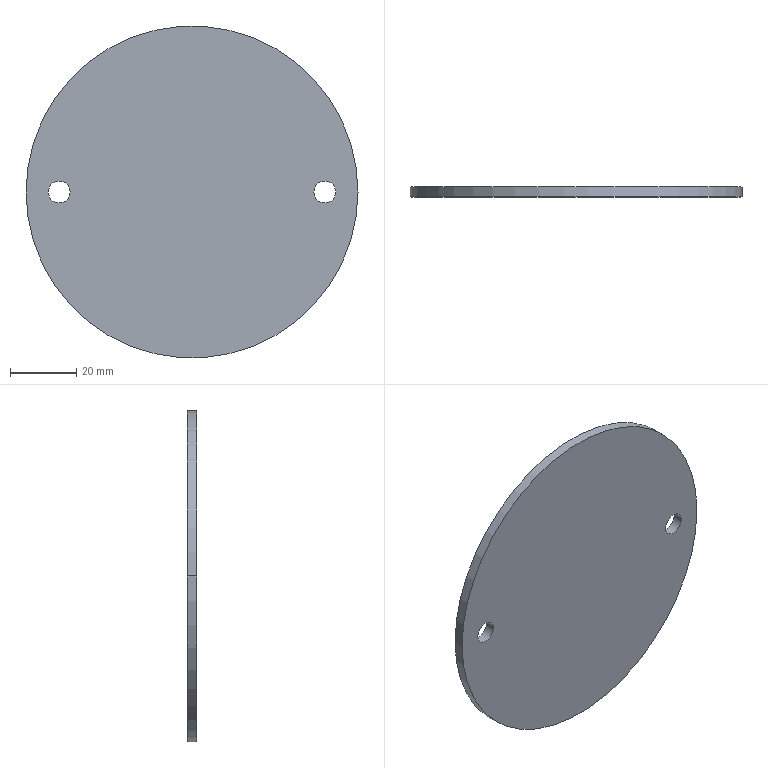Component | SolidWorks | YC1-250-04BalancerAssembly#16673-1_YC1-250-04-09Cover-1 | 1 solid | 8 faces | box 100 x 3 x 100 mm | volume 23357 mm3 | cylinder 6 | plane 2 | commonest cylinder face diameters 6.6 x4 100 x2 | material Plain Carbon Steel
STEP:
#1=COLOUR_RGB('',0.7922,0.8196,0.9333);
#2=FILL_AREA_STYLE_COLOUR('',#1);
#3=FILL_AREA_STYLE('',(#2));
#4=SURFACE_STYLE_FILL_AREA(#3);
#5=SURFACE_SIDE_STYLE('',(#4));
#6=SURFACE_STYLE_USAGE(.BOTH.,#5);
#7=PRESENTATION_STYLE_ASSIGNMENT((#6));
#8=CARTESIAN_POINT('',(-16.142,180.157,-0.));
#9=VERTEX_POINT('',#8);
#10=CARTESIAN_POINT('',(-20.079,180.157,-0.));
#11=VERTEX_POINT('',#10);
#12=CARTESIAN_POINT('',(-18.11,180.157,-0.));
#13=DIRECTION('',(-0.,1.,-0.));
#14=DIRECTION('',(-1.,0.,0.));
#15=AXIS2_PLACEMENT_3D('',#12,#13,#14);
#16=CIRCLE('',#15,1.969);
#17=EDGE_CURVE('',#9,#11,#16,.T.);
#18=ORIENTED_EDGE('',*,*,#17,.F.);
#19=CARTESIAN_POINT('',(-16.142,180.039,-0.));
#20=VERTEX_POINT('',#19);
#21=CARTESIAN_POINT('',(-16.142,180.157,-0.));
#22=DIRECTION('',(0.,-1.,0.));
#23=VECTOR('',#22,39.37);
#24=LINE('',#21,#23);
#25=EDGE_CURVE('',#9,#20,#24,.T.);
#26=ORIENTED_EDGE('',*,*,#25,.T.);
#27=CARTESIAN_POINT('',(-20.079,180.039,-0.));
#28=VERTEX_POINT('',#27);
#29=CARTESIAN_POINT('',(-18.11,180.039,-0.));
#30=DIRECTION('',(-0.,1.,-0.));
#31=DIRECTION('',(-1.,0.,0.));
#32=AXIS2_PLACEMENT_3D('',#29,#30,#31);
#33=CIRCLE('',#32,1.969);
#34=EDGE_CURVE('',#20,#28,#33,.T.);
#35=ORIENTED_EDGE('',*,*,#34,.T.);
#36=CARTESIAN_POINT('',(-20.079,180.157,-0.));
#37=DIRECTION('',(0.,-1.,0.));
#38=VECTOR('',#37,39.37);
#39=LINE('',#36,#38);
#40=EDGE_CURVE('',#11,#28,#39,.T.);
#41=ORIENTED_EDGE('',*,*,#40,.F.);
#42=EDGE_LOOP('',(#18,#26,#35,#41));
#43=FACE_OUTER_BOUND('',#42,.T.);
#44=CARTESIAN_POINT('',(-18.11,180.157,-0.));
#45=DIRECTION('',(0.,-1.,0.));
#46=DIRECTION('',(-1.,0.,0.));
#47=AXIS2_PLACEMENT_3D('',#44,#45,#46);
#48=CYLINDRICAL_SURFACE('',#47,1.969);
#49=ADVANCED_FACE('',(#43),#48,.T.);
#50=CARTESIAN_POINT('',(-16.665,180.039,-0.));
#51=VERTEX_POINT('',#50);
#52=CARTESIAN_POINT('',(-16.406,180.039,-0.));
#53=VERTEX_POINT('',#52);
#54=CARTESIAN_POINT('',(-16.535,180.039,-0.));
#55=DIRECTION('',(-0.,1.,-0.));
#56=DIRECTION('',(1.,0.,-0.));
#57=AXIS2_PLACEMENT_3D('',#54,#55,#56);
#58=CIRCLE('',#57,0.1299);
#59=EDGE_CURVE('',#51,#53,#58,.T.);
#60=ORIENTED_EDGE('',*,*,#59,.F.);
#61=CARTESIAN_POINT('',(-16.665,180.157,-0.));
#62=VERTEX_POINT('',#61);
#63=CARTESIAN_POINT('',(-16.665,180.157,-0.));
#64=DIRECTION('',(-0.,1.,-0.));
#65=VECTOR('',#64,39.37);
#66=LINE('',#63,#65);
#67=EDGE_CURVE('',#51,#62,#66,.T.);
#68=ORIENTED_EDGE('',*,*,#67,.T.);
#69=CARTESIAN_POINT('',(-16.406,180.157,-0.));
#70=VERTEX_POINT('',#69);
#71=CARTESIAN_POINT('',(-16.535,180.157,-0.));
#72=DIRECTION('',(0.,-1.,0.));
#73=DIRECTION('',(1.,0.,-0.));
#74=AXIS2_PLACEMENT_3D('',#71,#72,#73);
#75=CIRCLE('',#74,0.1299);
#76=EDGE_CURVE('',#70,#62,#75,.T.);
#77=ORIENTED_EDGE('',*,*,#76,.F.);
#78=CARTESIAN_POINT('',(-16.406,180.157,-0.));
#79=DIRECTION('',(-0.,1.,-0.));
#80=VECTOR('',#79,39.37);
#81=LINE('',#78,#80);
#82=EDGE_CURVE('',#53,#70,#81,.T.);
#83=ORIENTED_EDGE('',*,*,#82,.F.);
#84=EDGE_LOOP('',(#60,#68,#77,#83));
#85=FACE_OUTER_BOUND('',#84,.T.);
#86=CARTESIAN_POINT('',(-16.535,180.157,-0.));
#87=DIRECTION('',(-0.,1.,-0.));
#88=DIRECTION('',(1.,0.,-0.));
#89=AXIS2_PLACEMENT_3D('',#86,#87,#88);
#90=CYLINDRICAL_SURFACE('',#89,0.1299);
#91=ADVANCED_FACE('',(#85),#90,.F.);
#92=CARTESIAN_POINT('',(-19.815,180.039,-0.));
#93=VERTEX_POINT('',#92);
#94=CARTESIAN_POINT('',(-19.555,180.039,-0.));
#95=VERTEX_POINT('',#94);
#96=CARTESIAN_POINT('',(-19.685,180.039,-0.));
#97=DIRECTION('',(-0.,1.,-0.));
#98=DIRECTION('',(1.,0.,-0.));
#99=AXIS2_PLACEMENT_3D('',#96,#97,#98);
#100=CIRCLE('',#99,0.1299);
#101=EDGE_CURVE('',#93,#95,#100,.T.);
#102=ORIENTED_EDGE('',*,*,#101,.F.);
#103=CARTESIAN_POINT('',(-19.815,180.157,-0.));
#104=VERTEX_POINT('',#103);
#105=CARTESIAN_POINT('',(-19.815,180.157,-0.));
#106=DIRECTION('',(-0.,1.,-0.));
#107=VECTOR('',#106,39.37);
#108=LINE('',#105,#107);
#109=EDGE_CURVE('',#93,#104,#108,.T.);
#110=ORIENTED_EDGE('',*,*,#109,.T.);
#111=CARTESIAN_POINT('',(-19.555,180.157,-0.));
#112=VERTEX_POINT('',#111);
#113=CARTESIAN_POINT('',(-19.685,180.157,-0.));
#114=DIRECTION('',(0.,-1.,0.));
#115=DIRECTION('',(1.,0.,-0.));
#116=AXIS2_PLACEMENT_3D('',#113,#114,#115);
#117=CIRCLE('',#116,0.1299);
#118=EDGE_CURVE('',#112,#104,#117,.T.);
#119=ORIENTED_EDGE('',*,*,#118,.F.);
#120=CARTESIAN_POINT('',(-19.555,180.157,-0.));
#121=DIRECTION('',(-0.,1.,-0.));
#122=VECTOR('',#121,39.37);
#123=LINE('',#120,#122);
#124=EDGE_CURVE('',#95,#112,#123,.T.);
#125=ORIENTED_EDGE('',*,*,#124,.F.);
#126=EDGE_LOOP('',(#102,#110,#119,#125));
#127=FACE_OUTER_BOUND('',#126,.T.);
#128=CARTESIAN_POINT('',(-19.685,180.157,-0.));
#129=DIRECTION('',(-0.,1.,-0.));
#130=DIRECTION('',(1.,0.,-0.));
#131=AXIS2_PLACEMENT_3D('',#128,#129,#130);
#132=CYLINDRICAL_SURFACE('',#131,0.1299);
#133=ADVANCED_FACE('',(#127),#132,.F.);
#134=CARTESIAN_POINT('',(-18.11,180.157,-0.));
#135=DIRECTION('',(-0.,1.,-0.));
#136=DIRECTION('',(-1.,0.,0.));
#137=AXIS2_PLACEMENT_3D('',#134,#135,#136);
#138=CIRCLE('',#137,1.969);
#139=EDGE_CURVE('',#11,#9,#138,.T.);
#140=ORIENTED_EDGE('',*,*,#139,.T.);
#141=ORIENTED_EDGE('',*,*,#17,.T.);
#142=EDGE_LOOP('',(#140,#141));
#143=FACE_OUTER_BOUND('',#142,.T.);
#144=ORIENTED_EDGE('',*,*,#76,.T.);
#145=CARTESIAN_POINT('',(-16.535,180.157,-0.));
#146=DIRECTION('',(0.,-1.,0.));
#147=DIRECTION('',(1.,0.,-0.));
#148=AXIS2_PLACEMENT_3D('',#145,#146,#147);
#149=CIRCLE('',#148,0.1299);
#150=EDGE_CURVE('',#62,#70,#149,.T.);
#151=ORIENTED_EDGE('',*,*,#150,.T.);
#152=EDGE_LOOP('',(#144,#151));
#153=FACE_BOUND('',#152,.T.);
#154=ORIENTED_EDGE('',*,*,#118,.T.);
#155=CARTESIAN_POINT('',(-19.685,180.157,-0.));
#156=DIRECTION('',(0.,-1.,0.));
#157=DIRECTION('',(1.,0.,-0.));
#158=AXIS2_PLACEMENT_3D('',#155,#156,#157);
#159=CIRCLE('',#158,0.1299);
#160=EDGE_CURVE('',#104,#112,#159,.T.);
#161=ORIENTED_EDGE('',*,*,#160,.T.);
#162=EDGE_LOOP('',(#154,#161));
#163=FACE_BOUND('',#162,.T.);
#164=CARTESIAN_POINT('',(-18.11,180.157,-0.));
#165=DIRECTION('',(-0.,1.,-0.));
#166=DIRECTION('',(1.,0.,-0.));
#167=AXIS2_PLACEMENT_3D('',#164,#165,#166);
#168=PLANE('',#167);
#169=ADVANCED_FACE('',(#143,#153,#163),#168,.T.);
#170=ORIENTED_EDGE('',*,*,#25,.F.);
#171=ORIENTED_EDGE('',*,*,#139,.F.);
#172=ORIENTED_EDGE('',*,*,#40,.T.);
#173=CARTESIAN_POINT('',(-18.11,180.039,-0.));
#174=DIRECTION('',(-0.,1.,-0.));
#175=DIRECTION('',(-1.,0.,0.));
#176=AXIS2_PLACEMENT_3D('',#173,#174,#175);
#177=CIRCLE('',#176,1.969);
#178=EDGE_CURVE('',#28,#20,#177,.T.);
#179=ORIENTED_EDGE('',*,*,#178,.T.);
#180=EDGE_LOOP('',(#170,#171,#172,#179));
#181=FACE_OUTER_BOUND('',#180,.T.);
#182=CARTESIAN_POINT('',(-18.11,180.157,-0.));
#183=DIRECTION('',(0.,-1.,0.));
#184=DIRECTION('',(-1.,0.,0.));
#185=AXIS2_PLACEMENT_3D('',#182,#183,#184);
#186=CYLINDRICAL_SURFACE('',#185,1.969);
#187=ADVANCED_FACE('',(#181),#186,.T.);
#188=ORIENTED_EDGE('',*,*,#67,.F.);
#189=CARTESIAN_POINT('',(-16.535,180.039,-0.));
#190=DIRECTION('',(-0.,1.,-0.));
#191=DIRECTION('',(1.,0.,-0.));
#192=AXIS2_PLACEMENT_3D('',#189,#190,#191);
#193=CIRCLE('',#192,0.1299);
#194=EDGE_CURVE('',#53,#51,#193,.T.);
#195=ORIENTED_EDGE('',*,*,#194,.F.);
#196=ORIENTED_EDGE('',*,*,#82,.T.);
#197=ORIENTED_EDGE('',*,*,#150,.F.);
#198=EDGE_LOOP('',(#188,#195,#196,#197));
#199=FACE_OUTER_BOUND('',#198,.T.);
#200=CARTESIAN_POINT('',(-16.535,180.157,-0.));
#201=DIRECTION('',(-0.,1.,-0.));
#202=DIRECTION('',(1.,0.,-0.));
#203=AXIS2_PLACEMENT_3D('',#200,#201,#202);
#204=CYLINDRICAL_SURFACE('',#203,0.1299);
#205=ADVANCED_FACE('',(#199),#204,.F.);
#206=ORIENTED_EDGE('',*,*,#109,.F.);
#207=CARTESIAN_POINT('',(-19.685,180.039,-0.));
#208=DIRECTION('',(-0.,1.,-0.));
#209=DIRECTION('',(1.,0.,-0.));
#210=AXIS2_PLACEMENT_3D('',#207,#208,#209);
#211=CIRCLE('',#210,0.1299);
#212=EDGE_CURVE('',#95,#93,#211,.T.);
#213=ORIENTED_EDGE('',*,*,#212,.F.);
#214=ORIENTED_EDGE('',*,*,#124,.T.);
#215=ORIENTED_EDGE('',*,*,#160,.F.);
#216=EDGE_LOOP('',(#206,#213,#214,#215));
#217=FACE_OUTER_BOUND('',#216,.T.);
#218=CARTESIAN_POINT('',(-19.685,180.157,-0.));
#219=DIRECTION('',(-0.,1.,-0.));
#220=DIRECTION('',(1.,0.,-0.));
#221=AXIS2_PLACEMENT_3D('',#218,#219,#220);
#222=CYLINDRICAL_SURFACE('',#221,0.1299);
#223=ADVANCED_FACE('',(#217),#222,.F.);
#224=ORIENTED_EDGE('',*,*,#178,.F.);
#225=ORIENTED_EDGE('',*,*,#34,.F.);
#226=EDGE_LOOP('',(#224,#225));
#227=FACE_OUTER_BOUND('',#226,.T.);
#228=ORIENTED_EDGE('',*,*,#194,.T.);
#229=ORIENTED_EDGE('',*,*,#59,.T.);
#230=EDGE_LOOP('',(#228,#229));
#231=FACE_BOUND('',#230,.T.);
#232=ORIENTED_EDGE('',*,*,#212,.T.);
#233=ORIENTED_EDGE('',*,*,#101,.T.);
#234=EDGE_LOOP('',(#232,#233));
#235=FACE_BOUND('',#234,.T.);
#236=CARTESIAN_POINT('',(-18.11,180.039,-0.));
#237=DIRECTION('',(-0.,1.,-0.));
#238=DIRECTION('',(1.,0.,-0.));
#239=AXIS2_PLACEMENT_3D('',#236,#237,#238);
#240=PLANE('',#239);
#241=ADVANCED_FACE('',(#227,#231,#235),#240,.F.);
#242=CLOSED_SHELL('',(#49,#91,#133,#169,#187,#205,#223,#241));
#243=MANIFOLD_SOLID_BREP('',#242);
#244=STYLED_ITEM('',(#7),#243);
#245=PRESENTATION_LAYER_ASSIGNMENT('','',(#244));
#246=(LENGTH_UNIT()NAMED_UNIT(*)SI_UNIT($,.METRE.));
#247=LENGTH_MEASURE_WITH_UNIT(LENGTH_MEASURE(0.0254),#246);
#248=DIMENSIONAL_EXPONENTS(1.,0.,0.,0.,0.,0.,0.);
#249=(CONVERSION_BASED_UNIT('',#247)LENGTH_UNIT()NAMED_UNIT(#248));
#250=UNCERTAINTY_MEASURE_WITH_UNIT(LENGTH_MEASURE(0.00001),#249,'','');
#251=(NAMED_UNIT(*)PLANE_ANGLE_UNIT()SI_UNIT($,.RADIAN.));
#252=(NAMED_UNIT(*)SI_UNIT($,.STERADIAN.)SOLID_ANGLE_UNIT());
#253=(GEOMETRIC_REPRESENTATION_CONTEXT(3)GLOBAL_UNCERTAINTY_ASSIGNED_CONTEXT((#250))GLOBAL_UNIT_ASSIGNED_CONTEXT((#249,#251,#252))REPRESENTATION_CONTEXT('',''));
#254=MECHANICAL_DESIGN_GEOMETRIC_PRESENTATION_REPRESENTATION('',(#244),#253);
#255=CARTESIAN_POINT('',(0.,0.,0.));
#256=DIRECTION('',(0.,0.,1.));
#257=DIRECTION('',(1.,0.,0.));
#258=AXIS2_PLACEMENT_3D('',#255,#256,#257);
#259=(LENGTH_UNIT()NAMED_UNIT(*)SI_UNIT($,.METRE.));
#260=LENGTH_MEASURE_WITH_UNIT(LENGTH_MEASURE(0.0254),#259);
#261=DIMENSIONAL_EXPONENTS(1.,0.,0.,0.,0.,0.,0.);
#262=(CONVERSION_BASED_UNIT('',#260)LENGTH_UNIT()NAMED_UNIT(#261));
#263=UNCERTAINTY_MEASURE_WITH_UNIT(LENGTH_MEASURE(0.00001),#262,'','');
#264=(NAMED_UNIT(*)PLANE_ANGLE_UNIT()SI_UNIT($,.RADIAN.));
#265=(NAMED_UNIT(*)SI_UNIT($,.STERADIAN.)SOLID_ANGLE_UNIT());
#266=(GEOMETRIC_REPRESENTATION_CONTEXT(3)GLOBAL_UNCERTAINTY_ASSIGNED_CONTEXT((#263))GLOBAL_UNIT_ASSIGNED_CONTEXT((#262,#264,#265))REPRESENTATION_CONTEXT('',''));
#267=ADVANCED_BREP_SHAPE_REPRESENTATION('',(#243,#258),#266);